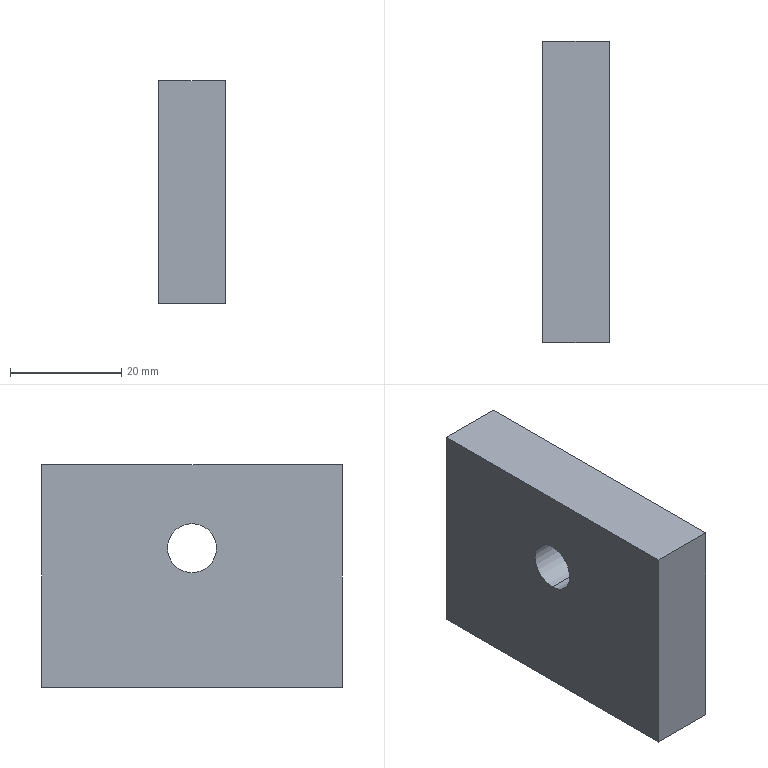Component | SolidWorks | CTM-HVS-52-OA-02-16-01-1 | 1 solid | 20 faces | box 12 x 54 x 40 mm | volume 24277 mm3 | cylinder 8 | cone 6 | plane 6 | commonest cylinder face diameters 5 x6 8.8 x2 | material Q235A
build123d program:
from build123d import *

# Parameters (mm, degrees)
SKETCH1_W               = 40
SKETCH1_H               = 54
EXTRUDE1_DEPTH          = 6
M10X1_25_TAPPED_HOLE1_D = 8.8
M6_TAPPED_HOLE1_D       = 5
M6_TAPPED_HOLE1_DEPTH   = 15
M6_TAPPED_HOLE1_TIP     = 1.502
M6_TAPPED_HOLE2_D       = 5
M6_TAPPED_HOLE2_DEPTH   = 15
M6_TAPPED_HOLE2_TIP     = 1.502


with BuildPart() as part:
    # Sketch1 → Extrude1 (new, symmetric)
    with BuildSketch(Plane.XY):
        Rectangle(SKETCH1_W, SKETCH1_H)
    extrude(amount=EXTRUDE1_DEPTH, both=True)

    # M10x1.25 Tapped Hole1 (through all)
    with Locations(Plane.XY.offset(6)):
        with Locations((5, 0)):
            Hole(M10X1_25_TAPPED_HOLE1_D / 2)

    # M6 Tapped Hole1
    with Locations(Plane.ZY.offset(20)):
        with Locations((0, 20), (0, -20)):
            Hole(M6_TAPPED_HOLE1_D / 2, depth=M6_TAPPED_HOLE1_DEPTH)
            with Locations((0, 0, -(M6_TAPPED_HOLE1_DEPTH + M6_TAPPED_HOLE1_TIP / 2))):  # 118° drill point
                Cone(0, M6_TAPPED_HOLE1_D / 2, M6_TAPPED_HOLE1_TIP, mode=Mode.SUBTRACT)

    # M6 Tapped Hole2
    with Locations(Plane(origin=(0, 27, 0), x_dir=(-1, 0, 0), z_dir=(0, 1, 0))):
        with Locations((-14, 0)):
            Hole(M6_TAPPED_HOLE2_D / 2, depth=M6_TAPPED_HOLE2_DEPTH)
            with Locations((0, 0, -(M6_TAPPED_HOLE2_DEPTH + M6_TAPPED_HOLE2_TIP / 2))):  # 118° drill point
                Cone(0, M6_TAPPED_HOLE2_D / 2, M6_TAPPED_HOLE2_TIP, mode=Mode.SUBTRACT)


solid = part.part

# Placed as in the assembly
solid = solid.moved(Location((223.693, 55.443, 25), (0, -90, 0)))
STEP:
#1=COLOUR_RGB('',0.7922,0.8196,0.9333);
#2=FILL_AREA_STYLE_COLOUR('',#1);
#3=FILL_AREA_STYLE('',(#2));
#4=SURFACE_STYLE_FILL_AREA(#3);
#5=SURFACE_SIDE_STYLE('',(#4));
#6=SURFACE_STYLE_USAGE(.BOTH.,#5);
#7=PRESENTATION_STYLE_ASSIGNMENT((#6));
#8=CARTESIAN_POINT('',(8.905,2.655,1.535));
#9=VERTEX_POINT('',#8);
#10=CARTESIAN_POINT('',(8.708,2.655,1.535));
#11=VERTEX_POINT('',#10);
#12=CARTESIAN_POINT('',(8.807,2.655,1.535));
#13=DIRECTION('',(-0.,1.,-0.));
#14=DIRECTION('',(-1.,0.,0.));
#15=AXIS2_PLACEMENT_3D('',#12,#13,#14);
#16=CIRCLE('',#15,0.09843);
#17=EDGE_CURVE('',#9,#11,#16,.T.);
#18=ORIENTED_EDGE('',*,*,#17,.F.);
#19=CARTESIAN_POINT('',(8.905,3.246,1.535));
#20=VERTEX_POINT('',#19);
#21=CARTESIAN_POINT('',(8.905,3.246,1.535));
#22=DIRECTION('',(-0.,1.,-0.));
#23=VECTOR('',#22,39.37);
#24=LINE('',#21,#23);
#25=EDGE_CURVE('',#9,#20,#24,.T.);
#26=ORIENTED_EDGE('',*,*,#25,.T.);
#27=CARTESIAN_POINT('',(8.708,3.246,1.535));
#28=VERTEX_POINT('',#27);
#29=CARTESIAN_POINT('',(8.807,3.246,1.535));
#30=DIRECTION('',(-0.,1.,-0.));
#31=DIRECTION('',(-1.,0.,0.));
#32=AXIS2_PLACEMENT_3D('',#29,#30,#31);
#33=CIRCLE('',#32,0.09843);
#34=EDGE_CURVE('',#20,#28,#33,.T.);
#35=ORIENTED_EDGE('',*,*,#34,.T.);
#36=CARTESIAN_POINT('',(8.708,3.246,1.535));
#37=DIRECTION('',(-0.,1.,-0.));
#38=VECTOR('',#37,39.37);
#39=LINE('',#36,#38);
#40=EDGE_CURVE('',#11,#28,#39,.T.);
#41=ORIENTED_EDGE('',*,*,#40,.F.);
#42=EDGE_LOOP('',(#18,#26,#35,#41));
#43=FACE_OUTER_BOUND('',#42,.T.);
#44=CARTESIAN_POINT('',(8.807,3.246,1.535));
#45=DIRECTION('',(-0.,1.,-0.));
#46=DIRECTION('',(-1.,0.,0.));
#47=AXIS2_PLACEMENT_3D('',#44,#45,#46);
#48=CYLINDRICAL_SURFACE('',#47,0.09843);
#49=ADVANCED_FACE('',(#43),#48,.F.);
#50=CARTESIAN_POINT('',(8.807,2.596,1.535));
#51=VERTEX_POINT('',#50);
#52=CARTESIAN_POINT('',(8.708,2.655,1.535));
#53=DIRECTION('',(-0.8572,0.515,-0.));
#54=VECTOR('',#53,39.37);
#55=LINE('',#52,#54);
#56=EDGE_CURVE('',#51,#11,#55,.T.);
#57=ORIENTED_EDGE('',*,*,#56,.F.);
#58=CARTESIAN_POINT('',(8.905,2.655,1.535));
#59=DIRECTION('',(0.8572,0.515,0.));
#60=VECTOR('',#59,39.37);
#61=LINE('',#58,#60);
#62=EDGE_CURVE('',#51,#9,#61,.T.);
#63=ORIENTED_EDGE('',*,*,#62,.T.);
#64=ORIENTED_EDGE('',*,*,#17,.T.);
#65=EDGE_LOOP('',(#57,#63,#64));
#66=FACE_OUTER_BOUND('',#65,.T.);
#67=CARTESIAN_POINT('',(8.807,2.655,1.535));
#68=DIRECTION('',(-0.,1.,-0.));
#69=DIRECTION('',(-1.,0.,0.));
#70=AXIS2_PLACEMENT_3D('',#67,#68,#69);
#71=CONICAL_SURFACE('',#70,0.09843,1.03);
#72=ADVANCED_FACE('',(#66),#71,.F.);
#73=CARTESIAN_POINT('',(8.905,2.97,0.7874));
#74=VERTEX_POINT('',#73);
#75=CARTESIAN_POINT('',(8.708,2.97,0.7874));
#76=VERTEX_POINT('',#75);
#77=CARTESIAN_POINT('',(8.807,2.97,0.7874));
#78=DIRECTION('',(0.,-0.,-1.));
#79=DIRECTION('',(-1.,0.,0.));
#80=AXIS2_PLACEMENT_3D('',#77,#78,#79);
#81=CIRCLE('',#80,0.09843);
#82=EDGE_CURVE('',#74,#76,#81,.T.);
#83=ORIENTED_EDGE('',*,*,#82,.F.);
#84=CARTESIAN_POINT('',(8.905,2.97,0.1969));
#85=VERTEX_POINT('',#84);
#86=CARTESIAN_POINT('',(8.905,2.97,0.1969));
#87=DIRECTION('',(0.,-0.,-1.));
#88=VECTOR('',#87,39.37);
#89=LINE('',#86,#88);
#90=EDGE_CURVE('',#74,#85,#89,.T.);
#91=ORIENTED_EDGE('',*,*,#90,.T.);
#92=CARTESIAN_POINT('',(8.708,2.97,0.1969));
#93=VERTEX_POINT('',#92);
#94=CARTESIAN_POINT('',(8.807,2.97,0.1969));
#95=DIRECTION('',(0.,-0.,-1.));
#96=DIRECTION('',(-1.,0.,0.));
#97=AXIS2_PLACEMENT_3D('',#94,#95,#96);
#98=CIRCLE('',#97,0.09843);
#99=EDGE_CURVE('',#85,#93,#98,.T.);
#100=ORIENTED_EDGE('',*,*,#99,.T.);
#101=CARTESIAN_POINT('',(8.708,2.97,0.1969));
#102=DIRECTION('',(0.,-0.,-1.));
#103=VECTOR('',#102,39.37);
#104=LINE('',#101,#103);
#105=EDGE_CURVE('',#76,#93,#104,.T.);
#106=ORIENTED_EDGE('',*,*,#105,.F.);
#107=EDGE_LOOP('',(#83,#91,#100,#106));
#108=FACE_OUTER_BOUND('',#107,.T.);
#109=CARTESIAN_POINT('',(8.807,2.97,0.1969));
#110=DIRECTION('',(0.,-0.,-1.));
#111=DIRECTION('',(-1.,0.,0.));
#112=AXIS2_PLACEMENT_3D('',#109,#110,#111);
#113=CYLINDRICAL_SURFACE('',#112,0.09843);
#114=ADVANCED_FACE('',(#108),#113,.F.);
#115=CARTESIAN_POINT('',(8.807,2.97,0.8465));
#116=VERTEX_POINT('',#115);
#117=CARTESIAN_POINT('',(8.708,2.97,0.7874));
#118=DIRECTION('',(-0.8572,-0.,-0.515));
#119=VECTOR('',#118,39.37);
#120=LINE('',#117,#119);
#121=EDGE_CURVE('',#116,#76,#120,.T.);
#122=ORIENTED_EDGE('',*,*,#121,.F.);
#123=CARTESIAN_POINT('',(8.905,2.97,0.7874));
#124=DIRECTION('',(0.8572,-0.,-0.515));
#125=VECTOR('',#124,39.37);
#126=LINE('',#123,#125);
#127=EDGE_CURVE('',#116,#74,#126,.T.);
#128=ORIENTED_EDGE('',*,*,#127,.T.);
#129=ORIENTED_EDGE('',*,*,#82,.T.);
#130=EDGE_LOOP('',(#122,#128,#129));
#131=FACE_OUTER_BOUND('',#130,.T.);
#132=CARTESIAN_POINT('',(8.807,2.97,0.7874));
#133=DIRECTION('',(0.,-0.,-1.));
#134=DIRECTION('',(-1.,0.,0.));
#135=AXIS2_PLACEMENT_3D('',#132,#133,#134);
#136=CONICAL_SURFACE('',#135,0.09843,1.03);
#137=ADVANCED_FACE('',(#131),#136,.F.);
#138=CARTESIAN_POINT('',(8.905,1.395,0.7874));
#139=VERTEX_POINT('',#138);
#140=CARTESIAN_POINT('',(8.708,1.395,0.7874));
#141=VERTEX_POINT('',#140);
#142=CARTESIAN_POINT('',(8.807,1.395,0.7874));
#143=DIRECTION('',(0.,-0.,-1.));
#144=DIRECTION('',(-1.,0.,0.));
#145=AXIS2_PLACEMENT_3D('',#142,#143,#144);
#146=CIRCLE('',#145,0.09843);
#147=EDGE_CURVE('',#139,#141,#146,.T.);
#148=ORIENTED_EDGE('',*,*,#147,.F.);
#149=CARTESIAN_POINT('',(8.905,1.395,0.1969));
#150=VERTEX_POINT('',#149);
#151=CARTESIAN_POINT('',(8.905,1.395,0.1969));
#152=DIRECTION('',(0.,-0.,-1.));
#153=VECTOR('',#152,39.37);
#154=LINE('',#151,#153);
#155=EDGE_CURVE('',#139,#150,#154,.T.);
#156=ORIENTED_EDGE('',*,*,#155,.T.);
#157=CARTESIAN_POINT('',(8.708,1.395,0.1969));
#158=VERTEX_POINT('',#157);
#159=CARTESIAN_POINT('',(8.807,1.395,0.1969));
#160=DIRECTION('',(0.,-0.,-1.));
#161=DIRECTION('',(-1.,0.,0.));
#162=AXIS2_PLACEMENT_3D('',#159,#160,#161);
#163=CIRCLE('',#162,0.09843);
#164=EDGE_CURVE('',#150,#158,#163,.T.);
#165=ORIENTED_EDGE('',*,*,#164,.T.);
#166=CARTESIAN_POINT('',(8.708,1.395,0.1969));
#167=DIRECTION('',(0.,-0.,-1.));
#168=VECTOR('',#167,39.37);
#169=LINE('',#166,#168);
#170=EDGE_CURVE('',#141,#158,#169,.T.);
#171=ORIENTED_EDGE('',*,*,#170,.F.);
#172=EDGE_LOOP('',(#148,#156,#165,#171));
#173=FACE_OUTER_BOUND('',#172,.T.);
#174=CARTESIAN_POINT('',(8.807,1.395,0.1969));
#175=DIRECTION('',(0.,-0.,-1.));
#176=DIRECTION('',(-1.,0.,0.));
#177=AXIS2_PLACEMENT_3D('',#174,#175,#176);
#178=CYLINDRICAL_SURFACE('',#177,0.09843);
#179=ADVANCED_FACE('',(#173),#178,.F.);
#180=CARTESIAN_POINT('',(8.807,1.395,0.8465));
#181=VERTEX_POINT('',#180);
#182=CARTESIAN_POINT('',(8.708,1.395,0.7874));
#183=DIRECTION('',(-0.8572,-0.,-0.515));
#184=VECTOR('',#183,39.37);
#185=LINE('',#182,#184);
#186=EDGE_CURVE('',#181,#141,#185,.T.);
#187=ORIENTED_EDGE('',*,*,#186,.F.);
#188=CARTESIAN_POINT('',(8.905,1.395,0.7874));
#189=DIRECTION('',(0.8572,-0.,-0.515));
#190=VECTOR('',#189,39.37);
#191=LINE('',#188,#190);
#192=EDGE_CURVE('',#181,#139,#191,.T.);
#193=ORIENTED_EDGE('',*,*,#192,.T.);
#194=ORIENTED_EDGE('',*,*,#147,.T.);
#195=EDGE_LOOP('',(#187,#193,#194));
#196=FACE_OUTER_BOUND('',#195,.T.);
#197=CARTESIAN_POINT('',(8.807,1.395,0.7874));
#198=DIRECTION('',(0.,-0.,-1.));
#199=DIRECTION('',(-1.,0.,0.));
#200=AXIS2_PLACEMENT_3D('',#197,#198,#199);
#201=CONICAL_SURFACE('',#200,0.09843,1.03);
#202=ADVANCED_FACE('',(#196),#201,.F.);
#203=CARTESIAN_POINT('',(9.043,2.183,1.008));
#204=VERTEX_POINT('',#203);
#205=CARTESIAN_POINT('',(9.043,2.183,1.354));
#206=VERTEX_POINT('',#205);
#207=CARTESIAN_POINT('',(9.043,2.183,1.181));
#208=DIRECTION('',(-1.,-0.,-0.));
#209=DIRECTION('',(0.,0.,1.));
#210=AXIS2_PLACEMENT_3D('',#207,#208,#209);
#211=CIRCLE('',#210,0.1732);
#212=EDGE_CURVE('',#204,#206,#211,.T.);
#213=ORIENTED_EDGE('',*,*,#212,.F.);
#214=CARTESIAN_POINT('',(8.571,2.183,1.008));
#215=VERTEX_POINT('',#214);
#216=CARTESIAN_POINT('',(8.571,2.183,1.008));
#217=DIRECTION('',(-1.,-0.,-0.));
#218=VECTOR('',#217,39.37);
#219=LINE('',#216,#218);
#220=EDGE_CURVE('',#204,#215,#219,.T.);
#221=ORIENTED_EDGE('',*,*,#220,.T.);
#222=CARTESIAN_POINT('',(8.571,2.183,1.354));
#223=VERTEX_POINT('',#222);
#224=CARTESIAN_POINT('',(8.571,2.183,1.181));
#225=DIRECTION('',(-1.,-0.,-0.));
#226=DIRECTION('',(0.,0.,1.));
#227=AXIS2_PLACEMENT_3D('',#224,#225,#226);
#228=CIRCLE('',#227,0.1732);
#229=EDGE_CURVE('',#215,#223,#228,.T.);
#230=ORIENTED_EDGE('',*,*,#229,.T.);
#231=CARTESIAN_POINT('',(8.571,2.183,1.354));
#232=DIRECTION('',(-1.,-0.,-0.));
#233=VECTOR('',#232,39.37);
#234=LINE('',#231,#233);
#235=EDGE_CURVE('',#206,#223,#234,.T.);
#236=ORIENTED_EDGE('',*,*,#235,.F.);
#237=EDGE_LOOP('',(#213,#221,#230,#236));
#238=FACE_OUTER_BOUND('',#237,.T.);
#239=CARTESIAN_POINT('',(8.571,2.183,1.181));
#240=DIRECTION('',(-1.,-0.,-0.));
#241=DIRECTION('',(0.,0.,1.));
#242=AXIS2_PLACEMENT_3D('',#239,#240,#241);
#243=CYLINDRICAL_SURFACE('',#242,0.1732);
#244=ADVANCED_FACE('',(#238),#243,.F.);
#245=CARTESIAN_POINT('',(9.043,1.12,1.772));
#246=VERTEX_POINT('',#245);
#247=CARTESIAN_POINT('',(9.043,3.246,1.772));
#248=VERTEX_POINT('',#247);
#249=CARTESIAN_POINT('',(9.043,3.246,1.772));
#250=DIRECTION('',(-0.,1.,-0.));
#251=VECTOR('',#250,39.37);
#252=LINE('',#249,#251);
#253=EDGE_CURVE('',#246,#248,#252,.T.);
#254=ORIENTED_EDGE('',*,*,#253,.T.);
#255=CARTESIAN_POINT('',(8.571,3.246,1.772));
#256=VERTEX_POINT('',#255);
#257=CARTESIAN_POINT('',(8.571,3.246,1.772));
#258=DIRECTION('',(1.,0.,0.));
#259=VECTOR('',#258,39.37);
#260=LINE('',#257,#259);
#261=EDGE_CURVE('',#256,#248,#260,.T.);
#262=ORIENTED_EDGE('',*,*,#261,.F.);
#263=CARTESIAN_POINT('',(8.571,1.12,1.772));
#264=VERTEX_POINT('',#263);
#265=CARTESIAN_POINT('',(8.571,3.246,1.772));
#266=DIRECTION('',(-0.,1.,-0.));
#267=VECTOR('',#266,39.37);
#268=LINE('',#265,#267);
#269=EDGE_CURVE('',#264,#256,#268,.T.);
#270=ORIENTED_EDGE('',*,*,#269,.F.);
#271=CARTESIAN_POINT('',(8.571,1.12,1.772));
#272=DIRECTION('',(1.,0.,0.));
#273=VECTOR('',#272,39.37);
#274=LINE('',#271,#273);
#275=EDGE_CURVE('',#264,#246,#274,.T.);
#276=ORIENTED_EDGE('',*,*,#275,.T.);
#277=EDGE_LOOP('',(#254,#262,#270,#276));
#278=FACE_OUTER_BOUND('',#277,.T.);
#279=CARTESIAN_POINT('',(8.571,3.246,1.772));
#280=DIRECTION('',(0.,-0.,-1.));
#281=DIRECTION('',(0.,-1.,0.));
#282=AXIS2_PLACEMENT_3D('',#279,#280,#281);
#283=PLANE('',#282);
#284=ADVANCED_FACE('',(#278),#283,.F.);
#285=CARTESIAN_POINT('',(8.807,3.246,1.535));
#286=DIRECTION('',(-0.,1.,-0.));
#287=DIRECTION('',(-1.,0.,0.));
#288=AXIS2_PLACEMENT_3D('',#285,#286,#287);
#289=CIRCLE('',#288,0.09843);
#290=EDGE_CURVE('',#28,#20,#289,.T.);
#291=ORIENTED_EDGE('',*,*,#290,.F.);
#292=ORIENTED_EDGE('',*,*,#34,.F.);
#293=EDGE_LOOP('',(#291,#292));
#294=FACE_BOUND('',#293,.T.);
#295=CARTESIAN_POINT('',(9.043,3.246,0.1969));
#296=VERTEX_POINT('',#295);
#297=CARTESIAN_POINT('',(9.043,3.246,0.1969));
#298=DIRECTION('',(0.,-0.,-1.));
#299=VECTOR('',#298,39.37);
#300=LINE('',#297,#299);
#301=EDGE_CURVE('',#248,#296,#300,.T.);
#302=ORIENTED_EDGE('',*,*,#301,.T.);
#303=CARTESIAN_POINT('',(8.571,3.246,0.1969));
#304=VERTEX_POINT('',#303);
#305=CARTESIAN_POINT('',(8.571,3.246,0.1969));
#306=DIRECTION('',(1.,0.,0.));
#307=VECTOR('',#306,39.37);
#308=LINE('',#305,#307);
#309=EDGE_CURVE('',#304,#296,#308,.T.);
#310=ORIENTED_EDGE('',*,*,#309,.F.);
#311=CARTESIAN_POINT('',(8.571,3.246,0.1969));
#312=DIRECTION('',(0.,-0.,-1.));
#313=VECTOR('',#312,39.37);
#314=LINE('',#311,#313);
#315=EDGE_CURVE('',#256,#304,#314,.T.);
#316=ORIENTED_EDGE('',*,*,#315,.F.);
#317=ORIENTED_EDGE('',*,*,#261,.T.);
#318=EDGE_LOOP('',(#302,#310,#316,#317));
#319=FACE_OUTER_BOUND('',#318,.T.);
#320=CARTESIAN_POINT('',(8.571,3.246,0.1969));
#321=DIRECTION('',(0.,-1.,0.));
#322=DIRECTION('',(1.,0.,0.));
#323=AXIS2_PLACEMENT_3D('',#320,#321,#322);
#324=PLANE('',#323);
#325=ADVANCED_FACE('',(#294,#319),#324,.F.);
#326=CARTESIAN_POINT('',(8.807,2.97,0.1969));
#327=DIRECTION('',(0.,-0.,-1.));
#328=DIRECTION('',(-1.,0.,0.));
#329=AXIS2_PLACEMENT_3D('',#326,#327,#328);
#330=CIRCLE('',#329,0.09843);
#331=EDGE_CURVE('',#93,#85,#330,.T.);
#332=ORIENTED_EDGE('',*,*,#331,.F.);
#333=ORIENTED_EDGE('',*,*,#99,.F.);
#334=EDGE_LOOP('',(#332,#333));
#335=FACE_BOUND('',#334,.T.);
#336=CARTESIAN_POINT('',(8.807,1.395,0.1969));
#337=DIRECTION('',(0.,-0.,-1.));
#338=DIRECTION('',(-1.,0.,0.));
#339=AXIS2_PLACEMENT_3D('',#336,#337,#338);
#340=CIRCLE('',#339,0.09843);
#341=EDGE_CURVE('',#158,#150,#340,.T.);
#342=ORIENTED_EDGE('',*,*,#341,.F.);
#343=ORIENTED_EDGE('',*,*,#164,.F.);
#344=EDGE_LOOP('',(#342,#343));
#345=FACE_BOUND('',#344,.T.);
#346=CARTESIAN_POINT('',(9.043,1.12,0.1969));
#347=VERTEX_POINT('',#346);
#348=CARTESIAN_POINT('',(9.043,3.246,0.1969));
#349=DIRECTION('',(0.,-1.,0.));
#350=VECTOR('',#349,39.37);
#351=LINE('',#348,#350);
#352=EDGE_CURVE('',#296,#347,#351,.T.);
#353=ORIENTED_EDGE('',*,*,#352,.T.);
#354=CARTESIAN_POINT('',(8.571,1.12,0.1969));
#355=VERTEX_POINT('',#354);
#356=CARTESIAN_POINT('',(8.571,1.12,0.1969));
#357=DIRECTION('',(1.,0.,0.));
#358=VECTOR('',#357,39.37);
#359=LINE('',#356,#358);
#360=EDGE_CURVE('',#355,#347,#359,.T.);
#361=ORIENTED_EDGE('',*,*,#360,.F.);
#362=CARTESIAN_POINT('',(8.571,3.246,0.1969));
#363=DIRECTION('',(0.,-1.,0.));
#364=VECTOR('',#363,39.37);
#365=LINE('',#362,#364);
#366=EDGE_CURVE('',#304,#355,#365,.T.);
#367=ORIENTED_EDGE('',*,*,#366,.F.);
#368=ORIENTED_EDGE('',*,*,#309,.T.);
#369=EDGE_LOOP('',(#353,#361,#367,#368));
#370=FACE_OUTER_BOUND('',#369,.T.);
#371=CARTESIAN_POINT('',(8.571,3.246,0.1969));
#372=DIRECTION('',(-0.,0.,1.));
#373=DIRECTION('',(-0.,1.,-0.));
#374=AXIS2_PLACEMENT_3D('',#371,#372,#373);
#375=PLANE('',#374);
#376=ADVANCED_FACE('',(#335,#345,#370),#375,.F.);
#377=CARTESIAN_POINT('',(9.043,1.12,0.1969));
#378=DIRECTION('',(-0.,0.,1.));
#379=VECTOR('',#378,39.37);
#380=LINE('',#377,#379);
#381=EDGE_CURVE('',#347,#246,#380,.T.);
#382=ORIENTED_EDGE('',*,*,#381,.T.);
#383=ORIENTED_EDGE('',*,*,#275,.F.);
#384=CARTESIAN_POINT('',(8.571,1.12,0.1969));
#385=DIRECTION('',(-0.,0.,1.));
#386=VECTOR('',#385,39.37);
#387=LINE('',#384,#386);
#388=EDGE_CURVE('',#355,#264,#387,.T.);
#389=ORIENTED_EDGE('',*,*,#388,.F.);
#390=ORIENTED_EDGE('',*,*,#360,.T.);
#391=EDGE_LOOP('',(#382,#383,#389,#390));
#392=FACE_OUTER_BOUND('',#391,.T.);
#393=CARTESIAN_POINT('',(8.571,1.12,0.1969));
#394=DIRECTION('',(-0.,1.,-0.));
#395=DIRECTION('',(-1.,-0.,-0.));
#396=AXIS2_PLACEMENT_3D('',#393,#394,#395);
#397=PLANE('',#396);
#398=ADVANCED_FACE('',(#392),#397,.F.);
#399=CARTESIAN_POINT('',(8.571,2.183,1.181));
#400=DIRECTION('',(-1.,-0.,-0.));
#401=DIRECTION('',(0.,0.,1.));
#402=AXIS2_PLACEMENT_3D('',#399,#400,#401);
#403=CIRCLE('',#402,0.1732);
#404=EDGE_CURVE('',#223,#215,#403,.T.);
#405=ORIENTED_EDGE('',*,*,#404,.F.);
#406=ORIENTED_EDGE('',*,*,#229,.F.);
#407=EDGE_LOOP('',(#405,#406));
#408=FACE_BOUND('',#407,.T.);
#409=ORIENTED_EDGE('',*,*,#269,.T.);
#410=ORIENTED_EDGE('',*,*,#315,.T.);
#411=ORIENTED_EDGE('',*,*,#366,.T.);
#412=ORIENTED_EDGE('',*,*,#388,.T.);
#413=EDGE_LOOP('',(#409,#410,#411,#412));
#414=FACE_OUTER_BOUND('',#413,.T.);
#415=CARTESIAN_POINT('',(8.571,1.12,1.772));
#416=DIRECTION('',(-1.,-0.,-0.));
#417=DIRECTION('',(-0.,0.,1.));
#418=AXIS2_PLACEMENT_3D('',#415,#416,#417);
#419=PLANE('',#418);
#420=ADVANCED_FACE('',(#408,#414),#419,.T.);
#421=CARTESIAN_POINT('',(9.043,2.183,1.181));
#422=DIRECTION('',(-1.,-0.,-0.));
#423=DIRECTION('',(0.,0.,1.));
#424=AXIS2_PLACEMENT_3D('',#421,#422,#423);
#425=CIRCLE('',#424,0.1732);
#426=EDGE_CURVE('',#206,#204,#425,.T.);
#427=ORIENTED_EDGE('',*,*,#426,.T.);
#428=ORIENTED_EDGE('',*,*,#212,.T.);
#429=EDGE_LOOP('',(#427,#428));
#430=FACE_BOUND('',#429,.T.);
#431=ORIENTED_EDGE('',*,*,#253,.F.);
#432=ORIENTED_EDGE('',*,*,#381,.F.);
#433=ORIENTED_EDGE('',*,*,#352,.F.);
#434=ORIENTED_EDGE('',*,*,#301,.F.);
#435=EDGE_LOOP('',(#431,#432,#433,#434));
#436=FACE_OUTER_BOUND('',#435,.T.);
#437=CARTESIAN_POINT('',(9.043,1.12,1.772));
#438=DIRECTION('',(-1.,-0.,-0.));
#439=DIRECTION('',(-0.,0.,1.));
#440=AXIS2_PLACEMENT_3D('',#437,#438,#439);
#441=PLANE('',#440);
#442=ADVANCED_FACE('',(#430,#436),#441,.F.);
#443=ORIENTED_EDGE('',*,*,#220,.F.);
#444=ORIENTED_EDGE('',*,*,#426,.F.);
#445=ORIENTED_EDGE('',*,*,#235,.T.);
#446=ORIENTED_EDGE('',*,*,#404,.T.);
#447=EDGE_LOOP('',(#443,#444,#445,#446));
#448=FACE_OUTER_BOUND('',#447,.T.);
#449=CARTESIAN_POINT('',(8.571,2.183,1.181));
#450=DIRECTION('',(-1.,-0.,-0.));
#451=DIRECTION('',(0.,0.,1.));
#452=AXIS2_PLACEMENT_3D('',#449,#450,#451);
#453=CYLINDRICAL_SURFACE('',#452,0.1732);
#454=ADVANCED_FACE('',(#448),#453,.F.);
#455=ORIENTED_EDGE('',*,*,#192,.F.);
#456=ORIENTED_EDGE('',*,*,#186,.T.);
#457=CARTESIAN_POINT('',(8.807,1.395,0.7874));
#458=DIRECTION('',(0.,-0.,-1.));
#459=DIRECTION('',(-1.,0.,0.));
#460=AXIS2_PLACEMENT_3D('',#457,#458,#459);
#461=CIRCLE('',#460,0.09843);
#462=EDGE_CURVE('',#141,#139,#461,.T.);
#463=ORIENTED_EDGE('',*,*,#462,.T.);
#464=EDGE_LOOP('',(#455,#456,#463));
#465=FACE_OUTER_BOUND('',#464,.T.);
#466=CARTESIAN_POINT('',(8.807,1.395,0.7874));
#467=DIRECTION('',(0.,-0.,-1.));
#468=DIRECTION('',(-1.,0.,0.));
#469=AXIS2_PLACEMENT_3D('',#466,#467,#468);
#470=CONICAL_SURFACE('',#469,0.09843,1.03);
#471=ADVANCED_FACE('',(#465),#470,.F.);
#472=ORIENTED_EDGE('',*,*,#155,.F.);
#473=ORIENTED_EDGE('',*,*,#462,.F.);
#474=ORIENTED_EDGE('',*,*,#170,.T.);
#475=ORIENTED_EDGE('',*,*,#341,.T.);
#476=EDGE_LOOP('',(#472,#473,#474,#475));
#477=FACE_OUTER_BOUND('',#476,.T.);
#478=CARTESIAN_POINT('',(8.807,1.395,0.1969));
#479=DIRECTION('',(0.,-0.,-1.));
#480=DIRECTION('',(-1.,0.,0.));
#481=AXIS2_PLACEMENT_3D('',#478,#479,#480);
#482=CYLINDRICAL_SURFACE('',#481,0.09843);
#483=ADVANCED_FACE('',(#477),#482,.F.);
#484=ORIENTED_EDGE('',*,*,#127,.F.);
#485=ORIENTED_EDGE('',*,*,#121,.T.);
#486=CARTESIAN_POINT('',(8.807,2.97,0.7874));
#487=DIRECTION('',(0.,-0.,-1.));
#488=DIRECTION('',(-1.,0.,0.));
#489=AXIS2_PLACEMENT_3D('',#486,#487,#488);
#490=CIRCLE('',#489,0.09843);
#491=EDGE_CURVE('',#76,#74,#490,.T.);
#492=ORIENTED_EDGE('',*,*,#491,.T.);
#493=EDGE_LOOP('',(#484,#485,#492));
#494=FACE_OUTER_BOUND('',#493,.T.);
#495=CARTESIAN_POINT('',(8.807,2.97,0.7874));
#496=DIRECTION('',(0.,-0.,-1.));
#497=DIRECTION('',(-1.,0.,0.));
#498=AXIS2_PLACEMENT_3D('',#495,#496,#497);
#499=CONICAL_SURFACE('',#498,0.09843,1.03);
#500=ADVANCED_FACE('',(#494),#499,.F.);
#501=ORIENTED_EDGE('',*,*,#90,.F.);
#502=ORIENTED_EDGE('',*,*,#491,.F.);
#503=ORIENTED_EDGE('',*,*,#105,.T.);
#504=ORIENTED_EDGE('',*,*,#331,.T.);
#505=EDGE_LOOP('',(#501,#502,#503,#504));
#506=FACE_OUTER_BOUND('',#505,.T.);
#507=CARTESIAN_POINT('',(8.807,2.97,0.1969));
#508=DIRECTION('',(0.,-0.,-1.));
#509=DIRECTION('',(-1.,0.,0.));
#510=AXIS2_PLACEMENT_3D('',#507,#508,#509);
#511=CYLINDRICAL_SURFACE('',#510,0.09843);
#512=ADVANCED_FACE('',(#506),#511,.F.);
#513=ORIENTED_EDGE('',*,*,#62,.F.);
#514=ORIENTED_EDGE('',*,*,#56,.T.);
#515=CARTESIAN_POINT('',(8.807,2.655,1.535));
#516=DIRECTION('',(-0.,1.,-0.));
#517=DIRECTION('',(-1.,0.,0.));
#518=AXIS2_PLACEMENT_3D('',#515,#516,#517);
#519=CIRCLE('',#518,0.09843);
#520=EDGE_CURVE('',#11,#9,#519,.T.);
#521=ORIENTED_EDGE('',*,*,#520,.T.);
#522=EDGE_LOOP('',(#513,#514,#521));
#523=FACE_OUTER_BOUND('',#522,.T.);
#524=CARTESIAN_POINT('',(8.807,2.655,1.535));
#525=DIRECTION('',(-0.,1.,-0.));
#526=DIRECTION('',(-1.,0.,0.));
#527=AXIS2_PLACEMENT_3D('',#524,#525,#526);
#528=CONICAL_SURFACE('',#527,0.09843,1.03);
#529=ADVANCED_FACE('',(#523),#528,.F.);
#530=ORIENTED_EDGE('',*,*,#25,.F.);
#531=ORIENTED_EDGE('',*,*,#520,.F.);
#532=ORIENTED_EDGE('',*,*,#40,.T.);
#533=ORIENTED_EDGE('',*,*,#290,.T.);
#534=EDGE_LOOP('',(#530,#531,#532,#533));
#535=FACE_OUTER_BOUND('',#534,.T.);
#536=CARTESIAN_POINT('',(8.807,3.246,1.535));
#537=DIRECTION('',(-0.,1.,-0.));
#538=DIRECTION('',(-1.,0.,0.));
#539=AXIS2_PLACEMENT_3D('',#536,#537,#538);
#540=CYLINDRICAL_SURFACE('',#539,0.09843);
#541=ADVANCED_FACE('',(#535),#540,.F.);
#542=CLOSED_SHELL('',(#49,#72,#114,#137,#179,#202,#244,#284,#325,#376,#398,#420,#442,#454,#471,#483,#500,#512,#529,#541));
#543=MANIFOLD_SOLID_BREP('',#542);
#544=STYLED_ITEM('',(#7),#543);
#545=PRESENTATION_LAYER_ASSIGNMENT('','',(#544));
#546=(LENGTH_UNIT()NAMED_UNIT(*)SI_UNIT($,.METRE.));
#547=LENGTH_MEASURE_WITH_UNIT(LENGTH_MEASURE(0.0254),#546);
#548=DIMENSIONAL_EXPONENTS(1.,0.,0.,0.,0.,0.,0.);
#549=(CONVERSION_BASED_UNIT('',#547)LENGTH_UNIT()NAMED_UNIT(#548));
#550=UNCERTAINTY_MEASURE_WITH_UNIT(LENGTH_MEASURE(0.00001),#549,'','');
#551=(NAMED_UNIT(*)PLANE_ANGLE_UNIT()SI_UNIT($,.RADIAN.));
#552=(NAMED_UNIT(*)SI_UNIT($,.STERADIAN.)SOLID_ANGLE_UNIT());
#553=(GEOMETRIC_REPRESENTATION_CONTEXT(3)GLOBAL_UNCERTAINTY_ASSIGNED_CONTEXT((#550))GLOBAL_UNIT_ASSIGNED_CONTEXT((#549,#551,#552))REPRESENTATION_CONTEXT('',''));
#554=MECHANICAL_DESIGN_GEOMETRIC_PRESENTATION_REPRESENTATION('',(#544),#553);
#555=CARTESIAN_POINT('',(0.,0.,0.));
#556=DIRECTION('',(0.,0.,1.));
#557=DIRECTION('',(1.,0.,0.));
#558=AXIS2_PLACEMENT_3D('',#555,#556,#557);
#559=(LENGTH_UNIT()NAMED_UNIT(*)SI_UNIT($,.METRE.));
#560=LENGTH_MEASURE_WITH_UNIT(LENGTH_MEASURE(0.0254),#559);
#561=DIMENSIONAL_EXPONENTS(1.,0.,0.,0.,0.,0.,0.);
#562=(CONVERSION_BASED_UNIT('',#560)LENGTH_UNIT()NAMED_UNIT(#561));
#563=UNCERTAINTY_MEASURE_WITH_UNIT(LENGTH_MEASURE(0.00001),#562,'','');
#564=(NAMED_UNIT(*)PLANE_ANGLE_UNIT()SI_UNIT($,.RADIAN.));
#565=(NAMED_UNIT(*)SI_UNIT($,.STERADIAN.)SOLID_ANGLE_UNIT());
#566=(GEOMETRIC_REPRESENTATION_CONTEXT(3)GLOBAL_UNCERTAINTY_ASSIGNED_CONTEXT((#563))GLOBAL_UNIT_ASSIGNED_CONTEXT((#562,#564,#565))REPRESENTATION_CONTEXT('',''));
#567=ADVANCED_BREP_SHAPE_REPRESENTATION('',(#543,#558),#566);